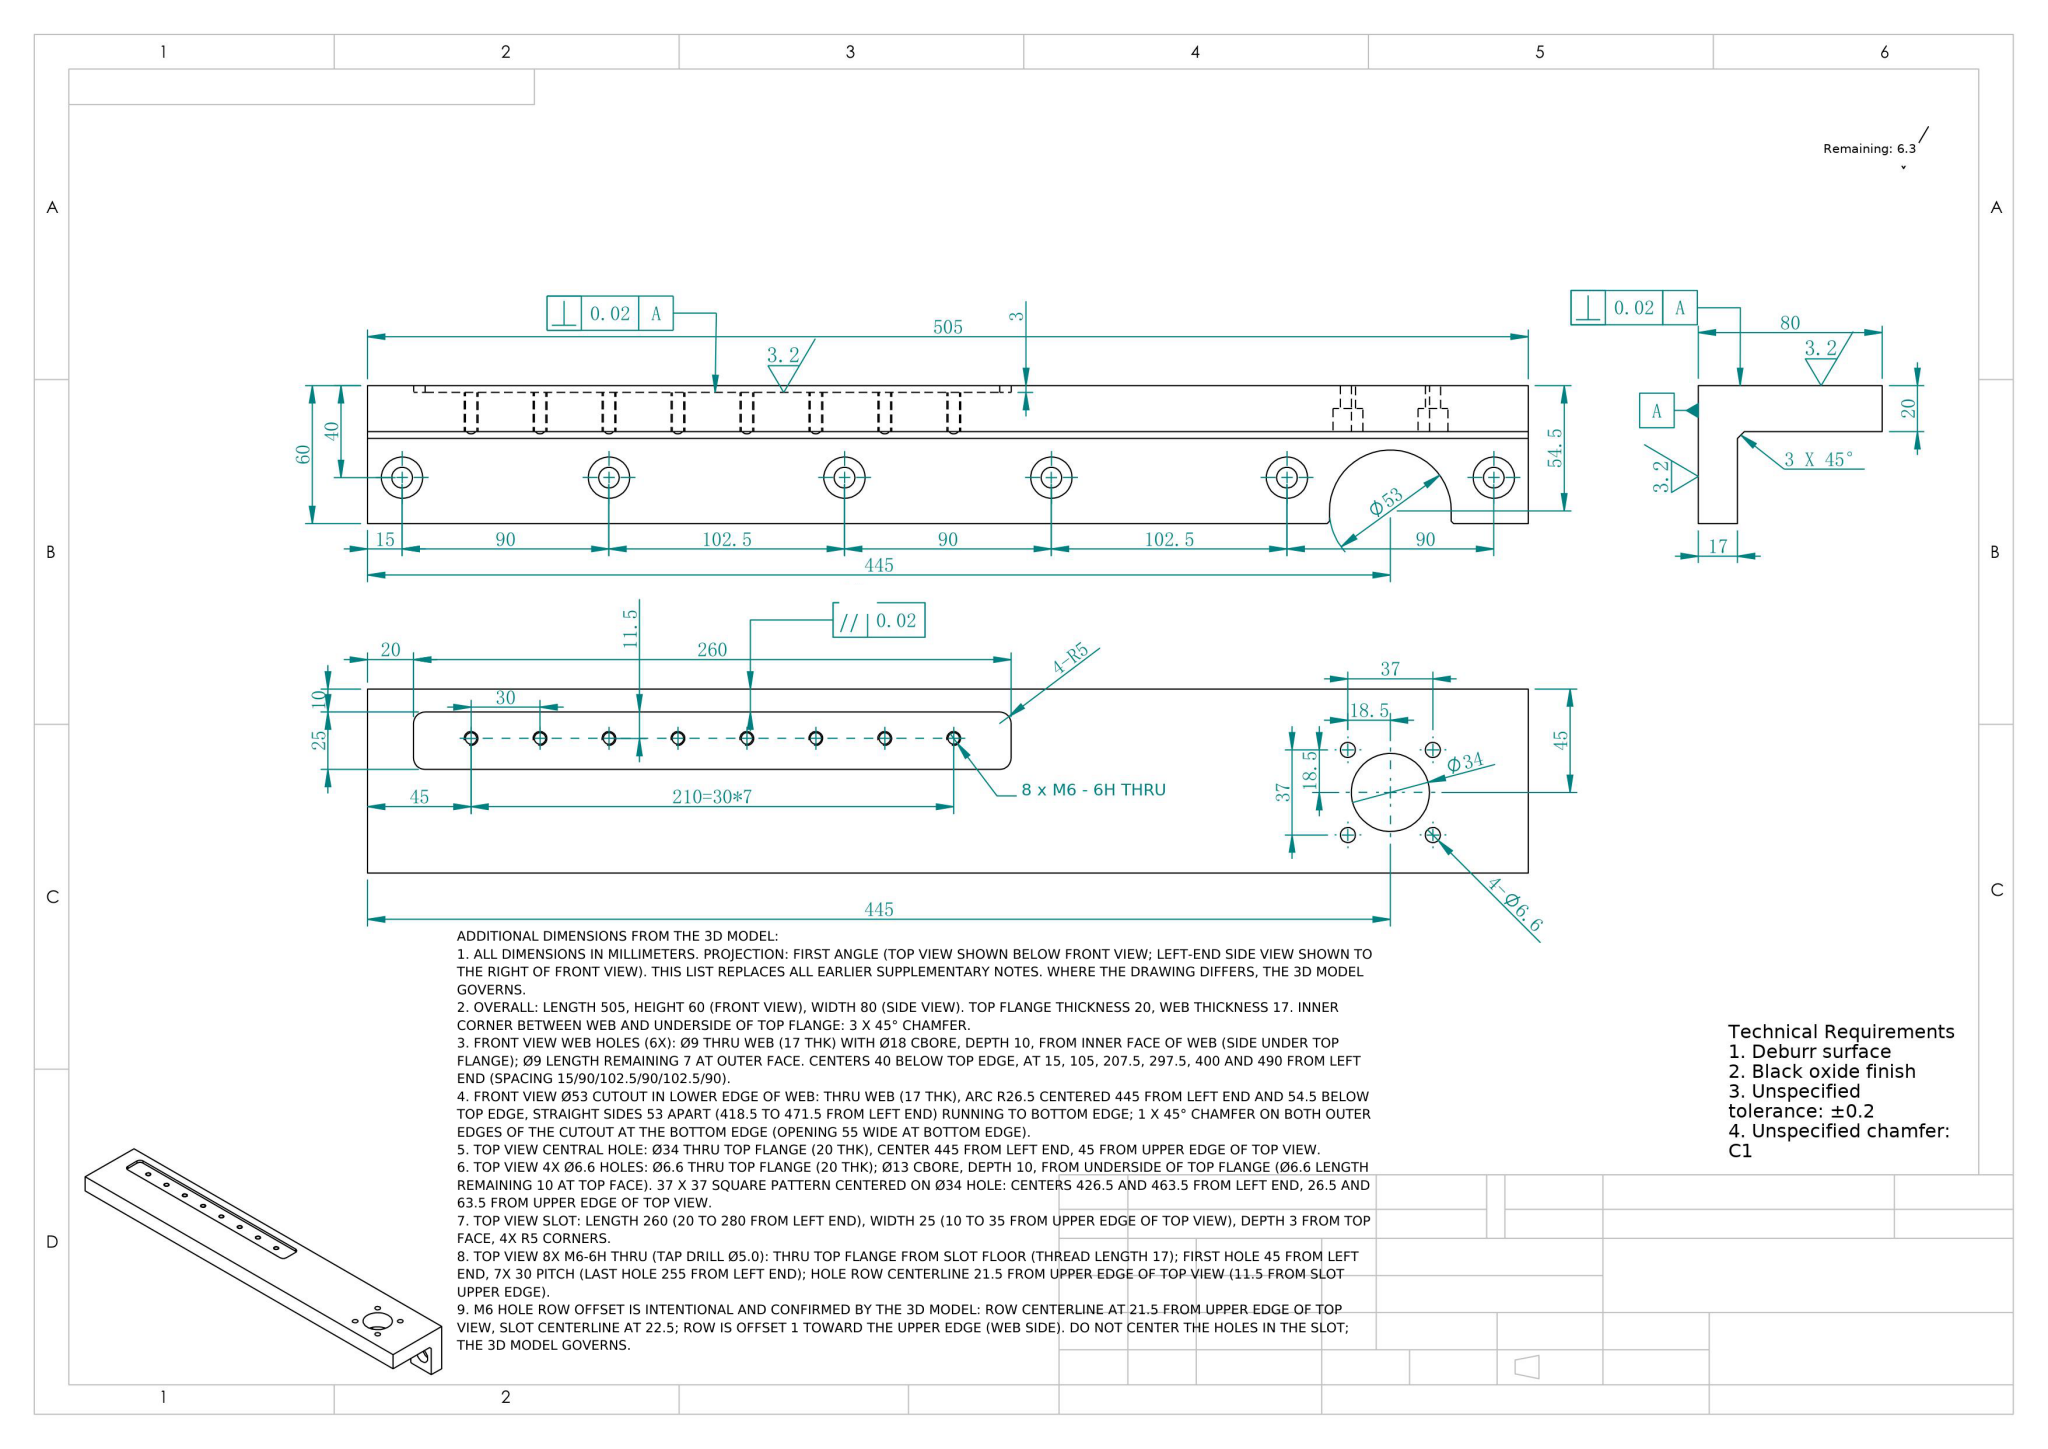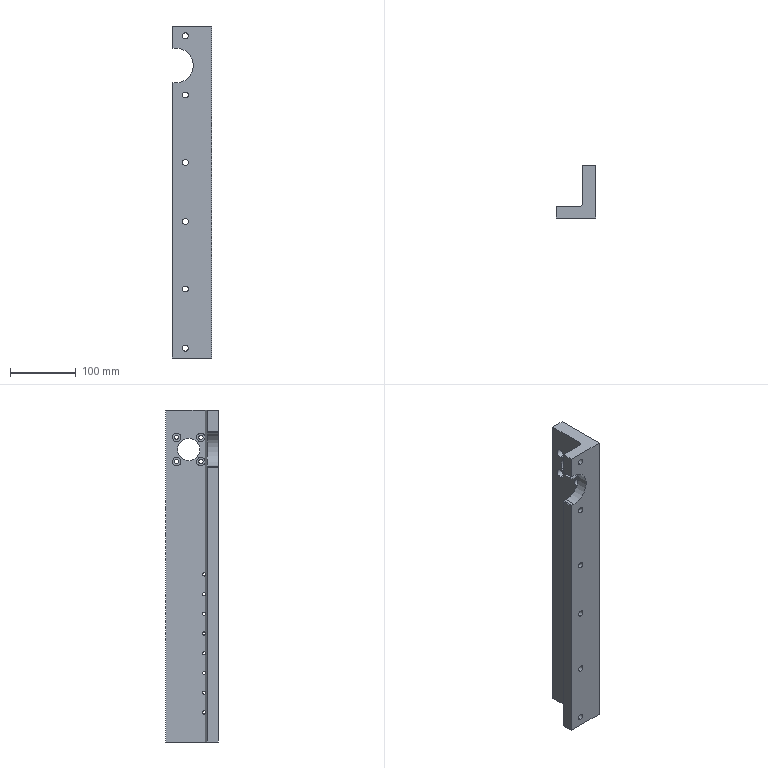Part | NX | mm | 1 solid | 92 faces | box 60 x 80 x 505 mm | volume 1065056 mm3 | cylinder 63 | plane 29 | commonest cylinder face diameters 5 x16 18 x12 9 x12 13 x8 6.6 x8 10 x4 34 x2 53 x1